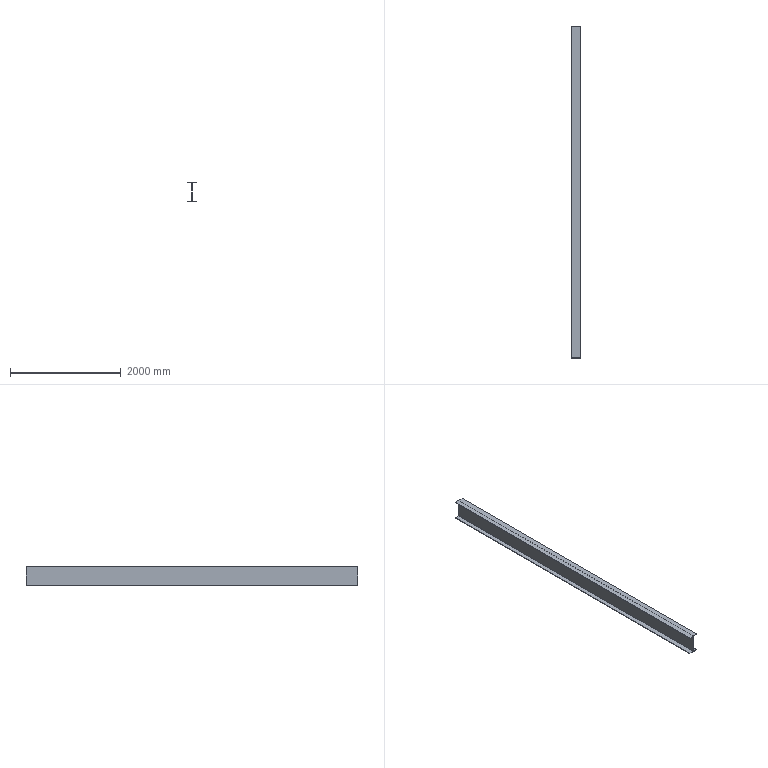Component | NX | ZHIJIA5 | 1 solid | 14 faces | box 175 x 6000 x 350 mm | volume 40800000 mm3 | plane 14
STEP:
#1=CARTESIAN_POINT('',(0.,0.,0.));
#2=DIRECTION('',(0.,0.,1.));
#3=DIRECTION('',(1.,0.,0.));
#4=AXIS2_PLACEMENT_3D('',#1,#2,#3);
#5=CARTESIAN_POINT('',(-2587.5,3000.,459.553));
#6=VERTEX_POINT('',#5);
#7=CARTESIAN_POINT('',(-2587.5,3000.,449.553));
#8=VERTEX_POINT('',#7);
#9=CARTESIAN_POINT('',(-2587.5,3000.,459.553));
#10=DIRECTION('',(-0.,0.,-1.));
#11=VECTOR('',#10,1.);
#12=LINE('',#9,#11);
#13=CARTESIAN_POINT('',(-2587.5,-3000.,459.553));
#14=DIRECTION('',(1.,0.,-0.));
#15=DIRECTION('',(0.,0.,1.));
#16=AXIS2_PLACEMENT_3D('',#13,#14,#15);
#17=PLANE('',#16);
#18=CARTESIAN_POINT('',(0.,-6000.));
#19=DIRECTION('',(-1.,0.));
#20=VECTOR('',#19,1.);
#21=LINE('',#18,#20);
#22=(GEOMETRIC_REPRESENTATION_CONTEXT(2)PARAMETRIC_REPRESENTATION_CONTEXT()REPRESENTATION_CONTEXT('',''));
#23=DEFINITIONAL_REPRESENTATION('',(#21),#22);
#24=PCURVE('',#17,#23);
#25=CARTESIAN_POINT('',(-2587.5,3000.,449.553));
#26=DIRECTION('',(0.,-1.,0.));
#27=DIRECTION('',(1.,0.,0.));
#28=AXIS2_PLACEMENT_3D('',#25,#26,#27);
#29=PLANE('',#28);
#30=CARTESIAN_POINT('',(0.,10.));
#31=DIRECTION('',(-0.,-1.));
#32=VECTOR('',#31,1.);
#33=LINE('',#30,#32);
#34=(GEOMETRIC_REPRESENTATION_CONTEXT(2)PARAMETRIC_REPRESENTATION_CONTEXT()REPRESENTATION_CONTEXT('',''));
#35=DEFINITIONAL_REPRESENTATION('',(#33),#34);
#36=PCURVE('',#29,#35);
#37=SURFACE_CURVE('',#12,(#24,#36),.PCURVE_S1.);
#38=EDGE_CURVE('',#6,#8,#37,.T.);
#39=ORIENTED_EDGE('',*,*,#38,.T.);
#40=CARTESIAN_POINT('',(-2587.5,-3000.,449.553));
#41=VERTEX_POINT('',#40);
#42=CARTESIAN_POINT('',(-2587.5,-3000.,449.553));
#43=DIRECTION('',(0.,1.,0.));
#44=VECTOR('',#43,1.);
#45=LINE('',#42,#44);
#46=CARTESIAN_POINT('',(-10.,0.));
#47=DIRECTION('',(0.,-1.));
#48=VECTOR('',#47,1.);
#49=LINE('',#46,#48);
#50=(GEOMETRIC_REPRESENTATION_CONTEXT(2)PARAMETRIC_REPRESENTATION_CONTEXT()REPRESENTATION_CONTEXT('',''));
#51=DEFINITIONAL_REPRESENTATION('',(#49),#50);
#52=PCURVE('',#17,#51);
#53=CARTESIAN_POINT('',(-2587.5,-3000.,449.553));
#54=DIRECTION('',(0.,0.,1.));
#55=DIRECTION('',(0.,-1.,0.));
#56=AXIS2_PLACEMENT_3D('',#53,#54,#55);
#57=PLANE('',#56);
#58=CARTESIAN_POINT('',(0.,0.));
#59=DIRECTION('',(-1.,0.));
#60=VECTOR('',#59,1.);
#61=LINE('',#58,#60);
#62=(GEOMETRIC_REPRESENTATION_CONTEXT(2)PARAMETRIC_REPRESENTATION_CONTEXT()REPRESENTATION_CONTEXT('',''));
#63=DEFINITIONAL_REPRESENTATION('',(#61),#62);
#64=PCURVE('',#57,#63);
#65=SURFACE_CURVE('',#45,(#52,#64),.PCURVE_S1.);
#66=EDGE_CURVE('',#41,#8,#65,.T.);
#67=ORIENTED_EDGE('',*,*,#66,.F.);
#68=CARTESIAN_POINT('',(-2587.5,-3000.,459.553));
#69=VERTEX_POINT('',#68);
#70=CARTESIAN_POINT('',(-2587.5,-3000.,459.553));
#71=DIRECTION('',(-0.,0.,-1.));
#72=VECTOR('',#71,1.);
#73=LINE('',#70,#72);
#74=CARTESIAN_POINT('',(0.,0.));
#75=DIRECTION('',(-1.,0.));
#76=VECTOR('',#75,1.);
#77=LINE('',#74,#76);
#78=(GEOMETRIC_REPRESENTATION_CONTEXT(2)PARAMETRIC_REPRESENTATION_CONTEXT()REPRESENTATION_CONTEXT('',''));
#79=DEFINITIONAL_REPRESENTATION('',(#77),#78);
#80=PCURVE('',#17,#79);
#81=CARTESIAN_POINT('',(-2587.5,-3000.,449.553));
#82=DIRECTION('',(0.,-1.,0.));
#83=DIRECTION('',(1.,0.,0.));
#84=AXIS2_PLACEMENT_3D('',#81,#82,#83);
#85=PLANE('',#84);
#86=CARTESIAN_POINT('',(0.,10.));
#87=DIRECTION('',(-0.,-1.));
#88=VECTOR('',#87,1.);
#89=LINE('',#86,#88);
#90=(GEOMETRIC_REPRESENTATION_CONTEXT(2)PARAMETRIC_REPRESENTATION_CONTEXT()REPRESENTATION_CONTEXT('',''));
#91=DEFINITIONAL_REPRESENTATION('',(#89),#90);
#92=PCURVE('',#85,#91);
#93=SURFACE_CURVE('',#73,(#80,#92),.PCURVE_S1.);
#94=EDGE_CURVE('',#69,#41,#93,.T.);
#95=ORIENTED_EDGE('',*,*,#94,.F.);
#96=CARTESIAN_POINT('',(-2587.5,-3000.,459.553));
#97=DIRECTION('',(0.,1.,0.));
#98=VECTOR('',#97,1.);
#99=LINE('',#96,#98);
#100=CARTESIAN_POINT('',(0.,0.));
#101=DIRECTION('',(0.,-1.));
#102=VECTOR('',#101,1.);
#103=LINE('',#100,#102);
#104=(GEOMETRIC_REPRESENTATION_CONTEXT(2)PARAMETRIC_REPRESENTATION_CONTEXT()REPRESENTATION_CONTEXT('',''));
#105=DEFINITIONAL_REPRESENTATION('',(#103),#104);
#106=PCURVE('',#17,#105);
#107=CARTESIAN_POINT('',(-2505.,-3000.,459.553));
#108=DIRECTION('',(0.,0.,-1.));
#109=DIRECTION('',(0.,1.,0.));
#110=AXIS2_PLACEMENT_3D('',#107,#108,#109);
#111=PLANE('',#110);
#112=CARTESIAN_POINT('',(0.,-82.5));
#113=DIRECTION('',(1.,0.));
#114=VECTOR('',#113,1.);
#115=LINE('',#112,#114);
#116=(GEOMETRIC_REPRESENTATION_CONTEXT(2)PARAMETRIC_REPRESENTATION_CONTEXT()REPRESENTATION_CONTEXT('',''));
#117=DEFINITIONAL_REPRESENTATION('',(#115),#116);
#118=PCURVE('',#111,#117);
#119=SURFACE_CURVE('',#99,(#106,#118),.PCURVE_S1.);
#120=EDGE_CURVE('',#69,#6,#119,.T.);
#121=ORIENTED_EDGE('',*,*,#120,.T.);
#122=EDGE_LOOP('',(#39,#67,#95,#121));
#123=FACE_BOUND('',#122,.T.);
#124=ADVANCED_FACE('',(#123),#17,.F.);
#125=CARTESIAN_POINT('',(-2412.5,3000.,449.553));
#126=VERTEX_POINT('',#125);
#127=CARTESIAN_POINT('',(-2587.5,3000.,449.553));
#128=DIRECTION('',(1.,0.,0.));
#129=VECTOR('',#128,1.);
#130=LINE('',#127,#129);
#131=CARTESIAN_POINT('',(-6000.,0.));
#132=DIRECTION('',(0.,1.));
#133=VECTOR('',#132,1.);
#134=LINE('',#131,#133);
#135=(GEOMETRIC_REPRESENTATION_CONTEXT(2)PARAMETRIC_REPRESENTATION_CONTEXT()REPRESENTATION_CONTEXT('',''));
#136=DEFINITIONAL_REPRESENTATION('',(#134),#135);
#137=PCURVE('',#57,#136);
#138=CARTESIAN_POINT('',(0.,0.));
#139=DIRECTION('',(1.,0.));
#140=VECTOR('',#139,1.);
#141=LINE('',#138,#140);
#142=(GEOMETRIC_REPRESENTATION_CONTEXT(2)PARAMETRIC_REPRESENTATION_CONTEXT()REPRESENTATION_CONTEXT('',''));
#143=DEFINITIONAL_REPRESENTATION('',(#141),#142);
#144=PCURVE('',#29,#143);
#145=SURFACE_CURVE('',#130,(#137,#144),.PCURVE_S1.);
#146=EDGE_CURVE('',#8,#126,#145,.T.);
#147=ORIENTED_EDGE('',*,*,#146,.T.);
#148=CARTESIAN_POINT('',(-2412.5,-3000.,449.553));
#149=VERTEX_POINT('',#148);
#150=CARTESIAN_POINT('',(-2412.5,-3000.,449.553));
#151=DIRECTION('',(0.,1.,0.));
#152=VECTOR('',#151,1.);
#153=LINE('',#150,#152);
#154=CARTESIAN_POINT('',(0.,175.));
#155=DIRECTION('',(-1.,0.));
#156=VECTOR('',#155,1.);
#157=LINE('',#154,#156);
#158=(GEOMETRIC_REPRESENTATION_CONTEXT(2)PARAMETRIC_REPRESENTATION_CONTEXT()REPRESENTATION_CONTEXT('',''));
#159=DEFINITIONAL_REPRESENTATION('',(#157),#158);
#160=PCURVE('',#57,#159);
#161=CARTESIAN_POINT('',(-2412.5,-3000.,449.553));
#162=DIRECTION('',(-1.,0.,0.));
#163=DIRECTION('',(-0.,0.,-1.));
#164=AXIS2_PLACEMENT_3D('',#161,#162,#163);
#165=PLANE('',#164);
#166=CARTESIAN_POINT('',(-0.,0.));
#167=DIRECTION('',(0.,-1.));
#168=VECTOR('',#167,1.);
#169=LINE('',#166,#168);
#170=(GEOMETRIC_REPRESENTATION_CONTEXT(2)PARAMETRIC_REPRESENTATION_CONTEXT()REPRESENTATION_CONTEXT('',''));
#171=DEFINITIONAL_REPRESENTATION('',(#169),#170);
#172=PCURVE('',#165,#171);
#173=SURFACE_CURVE('',#153,(#160,#172),.PCURVE_S1.);
#174=EDGE_CURVE('',#149,#126,#173,.T.);
#175=ORIENTED_EDGE('',*,*,#174,.F.);
#176=CARTESIAN_POINT('',(-2587.5,-3000.,449.553));
#177=DIRECTION('',(1.,0.,0.));
#178=VECTOR('',#177,1.);
#179=LINE('',#176,#178);
#180=CARTESIAN_POINT('',(0.,0.));
#181=DIRECTION('',(0.,1.));
#182=VECTOR('',#181,1.);
#183=LINE('',#180,#182);
#184=(GEOMETRIC_REPRESENTATION_CONTEXT(2)PARAMETRIC_REPRESENTATION_CONTEXT()REPRESENTATION_CONTEXT('',''));
#185=DEFINITIONAL_REPRESENTATION('',(#183),#184);
#186=PCURVE('',#57,#185);
#187=CARTESIAN_POINT('',(0.,0.));
#188=DIRECTION('',(1.,0.));
#189=VECTOR('',#188,1.);
#190=LINE('',#187,#189);
#191=(GEOMETRIC_REPRESENTATION_CONTEXT(2)PARAMETRIC_REPRESENTATION_CONTEXT()REPRESENTATION_CONTEXT('',''));
#192=DEFINITIONAL_REPRESENTATION('',(#190),#191);
#193=PCURVE('',#85,#192);
#194=SURFACE_CURVE('',#179,(#186,#193),.PCURVE_S1.);
#195=EDGE_CURVE('',#41,#149,#194,.T.);
#196=ORIENTED_EDGE('',*,*,#195,.F.);
#197=ORIENTED_EDGE('',*,*,#66,.T.);
#198=EDGE_LOOP('',(#147,#175,#196,#197));
#199=FACE_BOUND('',#198,.T.);
#200=ADVANCED_FACE('',(#199),#57,.F.);
#201=CARTESIAN_POINT('',(-2412.5,3000.,459.553));
#202=VERTEX_POINT('',#201);
#203=CARTESIAN_POINT('',(-2412.5,3000.,449.553));
#204=DIRECTION('',(0.,0.,1.));
#205=VECTOR('',#204,1.);
#206=LINE('',#203,#205);
#207=CARTESIAN_POINT('',(0.,-6000.));
#208=DIRECTION('',(-1.,0.));
#209=VECTOR('',#208,1.);
#210=LINE('',#207,#209);
#211=(GEOMETRIC_REPRESENTATION_CONTEXT(2)PARAMETRIC_REPRESENTATION_CONTEXT()REPRESENTATION_CONTEXT('',''));
#212=DEFINITIONAL_REPRESENTATION('',(#210),#211);
#213=PCURVE('',#165,#212);
#214=CARTESIAN_POINT('',(175.,-0.));
#215=DIRECTION('',(0.,1.));
#216=VECTOR('',#215,1.);
#217=LINE('',#214,#216);
#218=(GEOMETRIC_REPRESENTATION_CONTEXT(2)PARAMETRIC_REPRESENTATION_CONTEXT()REPRESENTATION_CONTEXT('',''));
#219=DEFINITIONAL_REPRESENTATION('',(#217),#218);
#220=PCURVE('',#29,#219);
#221=SURFACE_CURVE('',#206,(#213,#220),.PCURVE_S1.);
#222=EDGE_CURVE('',#126,#202,#221,.T.);
#223=ORIENTED_EDGE('',*,*,#222,.T.);
#224=CARTESIAN_POINT('',(-2412.5,-3000.,459.553));
#225=VERTEX_POINT('',#224);
#226=CARTESIAN_POINT('',(-2412.5,-3000.,459.553));
#227=DIRECTION('',(0.,1.,0.));
#228=VECTOR('',#227,1.);
#229=LINE('',#226,#228);
#230=CARTESIAN_POINT('',(-10.,0.));
#231=DIRECTION('',(0.,-1.));
#232=VECTOR('',#231,1.);
#233=LINE('',#230,#232);
#234=(GEOMETRIC_REPRESENTATION_CONTEXT(2)PARAMETRIC_REPRESENTATION_CONTEXT()REPRESENTATION_CONTEXT('',''));
#235=DEFINITIONAL_REPRESENTATION('',(#233),#234);
#236=PCURVE('',#165,#235);
#237=CARTESIAN_POINT('',(-2412.5,-3000.,459.553));
#238=DIRECTION('',(0.,0.,-1.));
#239=DIRECTION('',(0.,1.,0.));
#240=AXIS2_PLACEMENT_3D('',#237,#238,#239);
#241=PLANE('',#240);
#242=CARTESIAN_POINT('',(0.,0.));
#243=DIRECTION('',(1.,0.));
#244=VECTOR('',#243,1.);
#245=LINE('',#242,#244);
#246=(GEOMETRIC_REPRESENTATION_CONTEXT(2)PARAMETRIC_REPRESENTATION_CONTEXT()REPRESENTATION_CONTEXT('',''));
#247=DEFINITIONAL_REPRESENTATION('',(#245),#246);
#248=PCURVE('',#241,#247);
#249=SURFACE_CURVE('',#229,(#236,#248),.PCURVE_S1.);
#250=EDGE_CURVE('',#225,#202,#249,.T.);
#251=ORIENTED_EDGE('',*,*,#250,.F.);
#252=CARTESIAN_POINT('',(-2412.5,-3000.,449.553));
#253=DIRECTION('',(0.,0.,1.));
#254=VECTOR('',#253,1.);
#255=LINE('',#252,#254);
#256=CARTESIAN_POINT('',(0.,0.));
#257=DIRECTION('',(-1.,0.));
#258=VECTOR('',#257,1.);
#259=LINE('',#256,#258);
#260=(GEOMETRIC_REPRESENTATION_CONTEXT(2)PARAMETRIC_REPRESENTATION_CONTEXT()REPRESENTATION_CONTEXT('',''));
#261=DEFINITIONAL_REPRESENTATION('',(#259),#260);
#262=PCURVE('',#165,#261);
#263=CARTESIAN_POINT('',(175.,-0.));
#264=DIRECTION('',(0.,1.));
#265=VECTOR('',#264,1.);
#266=LINE('',#263,#265);
#267=(GEOMETRIC_REPRESENTATION_CONTEXT(2)PARAMETRIC_REPRESENTATION_CONTEXT()REPRESENTATION_CONTEXT('',''));
#268=DEFINITIONAL_REPRESENTATION('',(#266),#267);
#269=PCURVE('',#85,#268);
#270=SURFACE_CURVE('',#255,(#262,#269),.PCURVE_S1.);
#271=EDGE_CURVE('',#149,#225,#270,.T.);
#272=ORIENTED_EDGE('',*,*,#271,.F.);
#273=ORIENTED_EDGE('',*,*,#174,.T.);
#274=EDGE_LOOP('',(#223,#251,#272,#273));
#275=FACE_BOUND('',#274,.T.);
#276=ADVANCED_FACE('',(#275),#165,.F.);
#277=CARTESIAN_POINT('',(-2495.,3000.,459.553));
#278=VERTEX_POINT('',#277);
#279=CARTESIAN_POINT('',(-2412.5,3000.,459.553));
#280=DIRECTION('',(-1.,0.,0.));
#281=VECTOR('',#280,1.);
#282=LINE('',#279,#281);
#283=CARTESIAN_POINT('',(6000.,0.));
#284=DIRECTION('',(0.,-1.));
#285=VECTOR('',#284,1.);
#286=LINE('',#283,#285);
#287=(GEOMETRIC_REPRESENTATION_CONTEXT(2)PARAMETRIC_REPRESENTATION_CONTEXT()REPRESENTATION_CONTEXT('',''));
#288=DEFINITIONAL_REPRESENTATION('',(#286),#287);
#289=PCURVE('',#241,#288);
#290=CARTESIAN_POINT('',(175.,10.));
#291=DIRECTION('',(-1.,0.));
#292=VECTOR('',#291,1.);
#293=LINE('',#290,#292);
#294=(GEOMETRIC_REPRESENTATION_CONTEXT(2)PARAMETRIC_REPRESENTATION_CONTEXT()REPRESENTATION_CONTEXT('',''));
#295=DEFINITIONAL_REPRESENTATION('',(#293),#294);
#296=PCURVE('',#29,#295);
#297=SURFACE_CURVE('',#282,(#289,#296),.PCURVE_S1.);
#298=EDGE_CURVE('',#202,#278,#297,.T.);
#299=ORIENTED_EDGE('',*,*,#298,.T.);
#300=CARTESIAN_POINT('',(-2495.,-3000.,459.553));
#301=VERTEX_POINT('',#300);
#302=CARTESIAN_POINT('',(-2495.,-3000.,459.553));
#303=DIRECTION('',(0.,1.,0.));
#304=VECTOR('',#303,1.);
#305=LINE('',#302,#304);
#306=CARTESIAN_POINT('',(0.,-82.5));
#307=DIRECTION('',(1.,0.));
#308=VECTOR('',#307,1.);
#309=LINE('',#306,#308);
#310=(GEOMETRIC_REPRESENTATION_CONTEXT(2)PARAMETRIC_REPRESENTATION_CONTEXT()REPRESENTATION_CONTEXT('',''));
#311=DEFINITIONAL_REPRESENTATION('',(#309),#310);
#312=PCURVE('',#241,#311);
#313=CARTESIAN_POINT('',(-2495.,-3000.,459.553));
#314=DIRECTION('',(-1.,0.,0.));
#315=DIRECTION('',(-0.,0.,-1.));
#316=AXIS2_PLACEMENT_3D('',#313,#314,#315);
#317=PLANE('',#316);
#318=CARTESIAN_POINT('',(0.,0.));
#319=DIRECTION('',(0.,-1.));
#320=VECTOR('',#319,1.);
#321=LINE('',#318,#320);
#322=(GEOMETRIC_REPRESENTATION_CONTEXT(2)PARAMETRIC_REPRESENTATION_CONTEXT()REPRESENTATION_CONTEXT('',''));
#323=DEFINITIONAL_REPRESENTATION('',(#321),#322);
#324=PCURVE('',#317,#323);
#325=SURFACE_CURVE('',#305,(#312,#324),.PCURVE_S1.);
#326=EDGE_CURVE('',#301,#278,#325,.T.);
#327=ORIENTED_EDGE('',*,*,#326,.F.);
#328=CARTESIAN_POINT('',(-2412.5,-3000.,459.553));
#329=DIRECTION('',(-1.,0.,0.));
#330=VECTOR('',#329,1.);
#331=LINE('',#328,#330);
#332=CARTESIAN_POINT('',(0.,0.));
#333=DIRECTION('',(0.,-1.));
#334=VECTOR('',#333,1.);
#335=LINE('',#332,#334);
#336=(GEOMETRIC_REPRESENTATION_CONTEXT(2)PARAMETRIC_REPRESENTATION_CONTEXT()REPRESENTATION_CONTEXT('',''));
#337=DEFINITIONAL_REPRESENTATION('',(#335),#336);
#338=PCURVE('',#241,#337);
#339=CARTESIAN_POINT('',(175.,10.));
#340=DIRECTION('',(-1.,0.));
#341=VECTOR('',#340,1.);
#342=LINE('',#339,#341);
#343=(GEOMETRIC_REPRESENTATION_CONTEXT(2)PARAMETRIC_REPRESENTATION_CONTEXT()REPRESENTATION_CONTEXT('',''));
#344=DEFINITIONAL_REPRESENTATION('',(#342),#343);
#345=PCURVE('',#85,#344);
#346=SURFACE_CURVE('',#331,(#338,#345),.PCURVE_S1.);
#347=EDGE_CURVE('',#225,#301,#346,.T.);
#348=ORIENTED_EDGE('',*,*,#347,.F.);
#349=ORIENTED_EDGE('',*,*,#250,.T.);
#350=EDGE_LOOP('',(#299,#327,#348,#349));
#351=FACE_BOUND('',#350,.T.);
#352=ADVANCED_FACE('',(#351),#241,.F.);
#353=CARTESIAN_POINT('',(-2495.,3000.,789.553));
#354=VERTEX_POINT('',#353);
#355=CARTESIAN_POINT('',(-2495.,3000.,459.553));
#356=DIRECTION('',(0.,0.,1.));
#357=VECTOR('',#356,1.);
#358=LINE('',#355,#357);
#359=CARTESIAN_POINT('',(0.,-6000.));
#360=DIRECTION('',(-1.,0.));
#361=VECTOR('',#360,1.);
#362=LINE('',#359,#361);
#363=(GEOMETRIC_REPRESENTATION_CONTEXT(2)PARAMETRIC_REPRESENTATION_CONTEXT()REPRESENTATION_CONTEXT('',''));
#364=DEFINITIONAL_REPRESENTATION('',(#362),#363);
#365=PCURVE('',#317,#364);
#366=CARTESIAN_POINT('',(92.5,10.));
#367=DIRECTION('',(0.,1.));
#368=VECTOR('',#367,1.);
#369=LINE('',#366,#368);
#370=(GEOMETRIC_REPRESENTATION_CONTEXT(2)PARAMETRIC_REPRESENTATION_CONTEXT()REPRESENTATION_CONTEXT('',''));
#371=DEFINITIONAL_REPRESENTATION('',(#369),#370);
#372=PCURVE('',#29,#371);
#373=SURFACE_CURVE('',#358,(#365,#372),.PCURVE_S1.);
#374=EDGE_CURVE('',#278,#354,#373,.T.);
#375=ORIENTED_EDGE('',*,*,#374,.T.);
#376=CARTESIAN_POINT('',(-2495.,-3000.,789.553));
#377=VERTEX_POINT('',#376);
#378=CARTESIAN_POINT('',(-2495.,-3000.,789.553));
#379=DIRECTION('',(0.,1.,0.));
#380=VECTOR('',#379,1.);
#381=LINE('',#378,#380);
#382=CARTESIAN_POINT('',(-330.,0.));
#383=DIRECTION('',(0.,-1.));
#384=VECTOR('',#383,1.);
#385=LINE('',#382,#384);
#386=(GEOMETRIC_REPRESENTATION_CONTEXT(2)PARAMETRIC_REPRESENTATION_CONTEXT()REPRESENTATION_CONTEXT('',''));
#387=DEFINITIONAL_REPRESENTATION('',(#385),#386);
#388=PCURVE('',#317,#387);
#389=CARTESIAN_POINT('',(-2495.,-3000.,789.553));
#390=DIRECTION('',(0.,0.,1.));
#391=DIRECTION('',(0.,-1.,0.));
#392=AXIS2_PLACEMENT_3D('',#389,#390,#391);
#393=PLANE('',#392);
#394=CARTESIAN_POINT('',(0.,0.));
#395=DIRECTION('',(-1.,0.));
#396=VECTOR('',#395,1.);
#397=LINE('',#394,#396);
#398=(GEOMETRIC_REPRESENTATION_CONTEXT(2)PARAMETRIC_REPRESENTATION_CONTEXT()REPRESENTATION_CONTEXT('',''));
#399=DEFINITIONAL_REPRESENTATION('',(#397),#398);
#400=PCURVE('',#393,#399);
#401=SURFACE_CURVE('',#381,(#388,#400),.PCURVE_S1.);
#402=EDGE_CURVE('',#377,#354,#401,.T.);
#403=ORIENTED_EDGE('',*,*,#402,.F.);
#404=CARTESIAN_POINT('',(-2495.,-3000.,459.553));
#405=DIRECTION('',(0.,0.,1.));
#406=VECTOR('',#405,1.);
#407=LINE('',#404,#406);
#408=CARTESIAN_POINT('',(0.,0.));
#409=DIRECTION('',(-1.,0.));
#410=VECTOR('',#409,1.);
#411=LINE('',#408,#410);
#412=(GEOMETRIC_REPRESENTATION_CONTEXT(2)PARAMETRIC_REPRESENTATION_CONTEXT()REPRESENTATION_CONTEXT('',''));
#413=DEFINITIONAL_REPRESENTATION('',(#411),#412);
#414=PCURVE('',#317,#413);
#415=CARTESIAN_POINT('',(92.5,10.));
#416=DIRECTION('',(0.,1.));
#417=VECTOR('',#416,1.);
#418=LINE('',#415,#417);
#419=(GEOMETRIC_REPRESENTATION_CONTEXT(2)PARAMETRIC_REPRESENTATION_CONTEXT()REPRESENTATION_CONTEXT('',''));
#420=DEFINITIONAL_REPRESENTATION('',(#418),#419);
#421=PCURVE('',#85,#420);
#422=SURFACE_CURVE('',#407,(#414,#421),.PCURVE_S1.);
#423=EDGE_CURVE('',#301,#377,#422,.T.);
#424=ORIENTED_EDGE('',*,*,#423,.F.);
#425=ORIENTED_EDGE('',*,*,#326,.T.);
#426=EDGE_LOOP('',(#375,#403,#424,#425));
#427=FACE_BOUND('',#426,.T.);
#428=ADVANCED_FACE('',(#427),#317,.F.);
#429=CARTESIAN_POINT('',(-2412.5,3000.,789.553));
#430=VERTEX_POINT('',#429);
#431=CARTESIAN_POINT('',(-2495.,3000.,789.553));
#432=DIRECTION('',(1.,0.,0.));
#433=VECTOR('',#432,1.);
#434=LINE('',#431,#433);
#435=CARTESIAN_POINT('',(-6000.,0.));
#436=DIRECTION('',(0.,1.));
#437=VECTOR('',#436,1.);
#438=LINE('',#435,#437);
#439=(GEOMETRIC_REPRESENTATION_CONTEXT(2)PARAMETRIC_REPRESENTATION_CONTEXT()REPRESENTATION_CONTEXT('',''));
#440=DEFINITIONAL_REPRESENTATION('',(#438),#439);
#441=PCURVE('',#393,#440);
#442=CARTESIAN_POINT('',(92.5,340.));
#443=DIRECTION('',(1.,0.));
#444=VECTOR('',#443,1.);
#445=LINE('',#442,#444);
#446=(GEOMETRIC_REPRESENTATION_CONTEXT(2)PARAMETRIC_REPRESENTATION_CONTEXT()REPRESENTATION_CONTEXT('',''));
#447=DEFINITIONAL_REPRESENTATION('',(#445),#446);
#448=PCURVE('',#29,#447);
#449=SURFACE_CURVE('',#434,(#441,#448),.PCURVE_S1.);
#450=EDGE_CURVE('',#354,#430,#449,.T.);
#451=ORIENTED_EDGE('',*,*,#450,.T.);
#452=CARTESIAN_POINT('',(-2412.5,-3000.,789.553));
#453=VERTEX_POINT('',#452);
#454=CARTESIAN_POINT('',(-2412.5,-3000.,789.553));
#455=DIRECTION('',(0.,1.,0.));
#456=VECTOR('',#455,1.);
#457=LINE('',#454,#456);
#458=CARTESIAN_POINT('',(0.,82.5));
#459=DIRECTION('',(-1.,0.));
#460=VECTOR('',#459,1.);
#461=LINE('',#458,#460);
#462=(GEOMETRIC_REPRESENTATION_CONTEXT(2)PARAMETRIC_REPRESENTATION_CONTEXT()REPRESENTATION_CONTEXT('',''));
#463=DEFINITIONAL_REPRESENTATION('',(#461),#462);
#464=PCURVE('',#393,#463);
#465=CARTESIAN_POINT('',(-2412.5,-3000.,789.553));
#466=DIRECTION('',(-1.,0.,0.));
#467=DIRECTION('',(-0.,0.,-1.));
#468=AXIS2_PLACEMENT_3D('',#465,#466,#467);
#469=PLANE('',#468);
#470=CARTESIAN_POINT('',(0.,0.));
#471=DIRECTION('',(0.,-1.));
#472=VECTOR('',#471,1.);
#473=LINE('',#470,#472);
#474=(GEOMETRIC_REPRESENTATION_CONTEXT(2)PARAMETRIC_REPRESENTATION_CONTEXT()REPRESENTATION_CONTEXT('',''));
#475=DEFINITIONAL_REPRESENTATION('',(#473),#474);
#476=PCURVE('',#469,#475);
#477=SURFACE_CURVE('',#457,(#464,#476),.PCURVE_S1.);
#478=EDGE_CURVE('',#453,#430,#477,.T.);
#479=ORIENTED_EDGE('',*,*,#478,.F.);
#480=CARTESIAN_POINT('',(-2495.,-3000.,789.553));
#481=DIRECTION('',(1.,0.,0.));
#482=VECTOR('',#481,1.);
#483=LINE('',#480,#482);
#484=CARTESIAN_POINT('',(0.,0.));
#485=DIRECTION('',(0.,1.));
#486=VECTOR('',#485,1.);
#487=LINE('',#484,#486);
#488=(GEOMETRIC_REPRESENTATION_CONTEXT(2)PARAMETRIC_REPRESENTATION_CONTEXT()REPRESENTATION_CONTEXT('',''));
#489=DEFINITIONAL_REPRESENTATION('',(#487),#488);
#490=PCURVE('',#393,#489);
#491=CARTESIAN_POINT('',(92.5,340.));
#492=DIRECTION('',(1.,0.));
#493=VECTOR('',#492,1.);
#494=LINE('',#491,#493);
#495=(GEOMETRIC_REPRESENTATION_CONTEXT(2)PARAMETRIC_REPRESENTATION_CONTEXT()REPRESENTATION_CONTEXT('',''));
#496=DEFINITIONAL_REPRESENTATION('',(#494),#495);
#497=PCURVE('',#85,#496);
#498=SURFACE_CURVE('',#483,(#490,#497),.PCURVE_S1.);
#499=EDGE_CURVE('',#377,#453,#498,.T.);
#500=ORIENTED_EDGE('',*,*,#499,.F.);
#501=ORIENTED_EDGE('',*,*,#402,.T.);
#502=EDGE_LOOP('',(#451,#479,#500,#501));
#503=FACE_BOUND('',#502,.T.);
#504=ADVANCED_FACE('',(#503),#393,.F.);
#505=CARTESIAN_POINT('',(-2412.5,3000.,799.553));
#506=VERTEX_POINT('',#505);
#507=CARTESIAN_POINT('',(-2412.5,3000.,789.553));
#508=DIRECTION('',(0.,0.,1.));
#509=VECTOR('',#508,1.);
#510=LINE('',#507,#509);
#511=CARTESIAN_POINT('',(0.,-6000.));
#512=DIRECTION('',(-1.,0.));
#513=VECTOR('',#512,1.);
#514=LINE('',#511,#513);
#515=(GEOMETRIC_REPRESENTATION_CONTEXT(2)PARAMETRIC_REPRESENTATION_CONTEXT()REPRESENTATION_CONTEXT('',''));
#516=DEFINITIONAL_REPRESENTATION('',(#514),#515);
#517=PCURVE('',#469,#516);
#518=CARTESIAN_POINT('',(175.,340.));
#519=DIRECTION('',(0.,1.));
#520=VECTOR('',#519,1.);
#521=LINE('',#518,#520);
#522=(GEOMETRIC_REPRESENTATION_CONTEXT(2)PARAMETRIC_REPRESENTATION_CONTEXT()REPRESENTATION_CONTEXT('',''));
#523=DEFINITIONAL_REPRESENTATION('',(#521),#522);
#524=PCURVE('',#29,#523);
#525=SURFACE_CURVE('',#510,(#517,#524),.PCURVE_S1.);
#526=EDGE_CURVE('',#430,#506,#525,.T.);
#527=ORIENTED_EDGE('',*,*,#526,.T.);
#528=CARTESIAN_POINT('',(-2412.5,-3000.,799.553));
#529=VERTEX_POINT('',#528);
#530=CARTESIAN_POINT('',(-2412.5,-3000.,799.553));
#531=DIRECTION('',(0.,1.,0.));
#532=VECTOR('',#531,1.);
#533=LINE('',#530,#532);
#534=CARTESIAN_POINT('',(-10.,0.));
#535=DIRECTION('',(0.,-1.));
#536=VECTOR('',#535,1.);
#537=LINE('',#534,#536);
#538=(GEOMETRIC_REPRESENTATION_CONTEXT(2)PARAMETRIC_REPRESENTATION_CONTEXT()REPRESENTATION_CONTEXT('',''));
#539=DEFINITIONAL_REPRESENTATION('',(#537),#538);
#540=PCURVE('',#469,#539);
#541=CARTESIAN_POINT('',(-2412.5,-3000.,799.553));
#542=DIRECTION('',(0.,0.,-1.));
#543=DIRECTION('',(0.,1.,0.));
#544=AXIS2_PLACEMENT_3D('',#541,#542,#543);
#545=PLANE('',#544);
#546=CARTESIAN_POINT('',(0.,0.));
#547=DIRECTION('',(1.,0.));
#548=VECTOR('',#547,1.);
#549=LINE('',#546,#548);
#550=(GEOMETRIC_REPRESENTATION_CONTEXT(2)PARAMETRIC_REPRESENTATION_CONTEXT()REPRESENTATION_CONTEXT('',''));
#551=DEFINITIONAL_REPRESENTATION('',(#549),#550);
#552=PCURVE('',#545,#551);
#553=SURFACE_CURVE('',#533,(#540,#552),.PCURVE_S1.);
#554=EDGE_CURVE('',#529,#506,#553,.T.);
#555=ORIENTED_EDGE('',*,*,#554,.F.);
#556=CARTESIAN_POINT('',(-2412.5,-3000.,789.553));
#557=DIRECTION('',(0.,0.,1.));
#558=VECTOR('',#557,1.);
#559=LINE('',#556,#558);
#560=CARTESIAN_POINT('',(0.,0.));
#561=DIRECTION('',(-1.,0.));
#562=VECTOR('',#561,1.);
#563=LINE('',#560,#562);
#564=(GEOMETRIC_REPRESENTATION_CONTEXT(2)PARAMETRIC_REPRESENTATION_CONTEXT()REPRESENTATION_CONTEXT('',''));
#565=DEFINITIONAL_REPRESENTATION('',(#563),#564);
#566=PCURVE('',#469,#565);
#567=CARTESIAN_POINT('',(175.,340.));
#568=DIRECTION('',(0.,1.));
#569=VECTOR('',#568,1.);
#570=LINE('',#567,#569);
#571=(GEOMETRIC_REPRESENTATION_CONTEXT(2)PARAMETRIC_REPRESENTATION_CONTEXT()REPRESENTATION_CONTEXT('',''));
#572=DEFINITIONAL_REPRESENTATION('',(#570),#571);
#573=PCURVE('',#85,#572);
#574=SURFACE_CURVE('',#559,(#566,#573),.PCURVE_S1.);
#575=EDGE_CURVE('',#453,#529,#574,.T.);
#576=ORIENTED_EDGE('',*,*,#575,.F.);
#577=ORIENTED_EDGE('',*,*,#478,.T.);
#578=EDGE_LOOP('',(#527,#555,#576,#577));
#579=FACE_BOUND('',#578,.T.);
#580=ADVANCED_FACE('',(#579),#469,.F.);
#581=CARTESIAN_POINT('',(-2587.5,3000.,799.553));
#582=VERTEX_POINT('',#581);
#583=CARTESIAN_POINT('',(-2412.5,3000.,799.553));
#584=DIRECTION('',(-1.,0.,0.));
#585=VECTOR('',#584,1.);
#586=LINE('',#583,#585);
#587=CARTESIAN_POINT('',(6000.,0.));
#588=DIRECTION('',(0.,-1.));
#589=VECTOR('',#588,1.);
#590=LINE('',#587,#589);
#591=(GEOMETRIC_REPRESENTATION_CONTEXT(2)PARAMETRIC_REPRESENTATION_CONTEXT()REPRESENTATION_CONTEXT('',''));
#592=DEFINITIONAL_REPRESENTATION('',(#590),#591);
#593=PCURVE('',#545,#592);
#594=CARTESIAN_POINT('',(175.,350.));
#595=DIRECTION('',(-1.,0.));
#596=VECTOR('',#595,1.);
#597=LINE('',#594,#596);
#598=(GEOMETRIC_REPRESENTATION_CONTEXT(2)PARAMETRIC_REPRESENTATION_CONTEXT()REPRESENTATION_CONTEXT('',''));
#599=DEFINITIONAL_REPRESENTATION('',(#597),#598);
#600=PCURVE('',#29,#599);
#601=SURFACE_CURVE('',#586,(#593,#600),.PCURVE_S1.);
#602=EDGE_CURVE('',#506,#582,#601,.T.);
#603=ORIENTED_EDGE('',*,*,#602,.T.);
#604=CARTESIAN_POINT('',(-2587.5,-3000.,799.553));
#605=VERTEX_POINT('',#604);
#606=CARTESIAN_POINT('',(-2587.5,-3000.,799.553));
#607=DIRECTION('',(0.,1.,0.));
#608=VECTOR('',#607,1.);
#609=LINE('',#606,#608);
#610=CARTESIAN_POINT('',(0.,-175.));
#611=DIRECTION('',(1.,0.));
#612=VECTOR('',#611,1.);
#613=LINE('',#610,#612);
#614=(GEOMETRIC_REPRESENTATION_CONTEXT(2)PARAMETRIC_REPRESENTATION_CONTEXT()REPRESENTATION_CONTEXT('',''));
#615=DEFINITIONAL_REPRESENTATION('',(#613),#614);
#616=PCURVE('',#545,#615);
#617=CARTESIAN_POINT('',(-2587.5,-3000.,799.553));
#618=DIRECTION('',(1.,0.,-0.));
#619=DIRECTION('',(0.,0.,1.));
#620=AXIS2_PLACEMENT_3D('',#617,#618,#619);
#621=PLANE('',#620);
#622=CARTESIAN_POINT('',(0.,0.));
#623=DIRECTION('',(0.,-1.));
#624=VECTOR('',#623,1.);
#625=LINE('',#622,#624);
#626=(GEOMETRIC_REPRESENTATION_CONTEXT(2)PARAMETRIC_REPRESENTATION_CONTEXT()REPRESENTATION_CONTEXT('',''));
#627=DEFINITIONAL_REPRESENTATION('',(#625),#626);
#628=PCURVE('',#621,#627);
#629=SURFACE_CURVE('',#609,(#616,#628),.PCURVE_S1.);
#630=EDGE_CURVE('',#605,#582,#629,.T.);
#631=ORIENTED_EDGE('',*,*,#630,.F.);
#632=CARTESIAN_POINT('',(-2412.5,-3000.,799.553));
#633=DIRECTION('',(-1.,0.,0.));
#634=VECTOR('',#633,1.);
#635=LINE('',#632,#634);
#636=CARTESIAN_POINT('',(0.,0.));
#637=DIRECTION('',(0.,-1.));
#638=VECTOR('',#637,1.);
#639=LINE('',#636,#638);
#640=(GEOMETRIC_REPRESENTATION_CONTEXT(2)PARAMETRIC_REPRESENTATION_CONTEXT()REPRESENTATION_CONTEXT('',''));
#641=DEFINITIONAL_REPRESENTATION('',(#639),#640);
#642=PCURVE('',#545,#641);
#643=CARTESIAN_POINT('',(175.,350.));
#644=DIRECTION('',(-1.,0.));
#645=VECTOR('',#644,1.);
#646=LINE('',#643,#645);
#647=(GEOMETRIC_REPRESENTATION_CONTEXT(2)PARAMETRIC_REPRESENTATION_CONTEXT()REPRESENTATION_CONTEXT('',''));
#648=DEFINITIONAL_REPRESENTATION('',(#646),#647);
#649=PCURVE('',#85,#648);
#650=SURFACE_CURVE('',#635,(#642,#649),.PCURVE_S1.);
#651=EDGE_CURVE('',#529,#605,#650,.T.);
#652=ORIENTED_EDGE('',*,*,#651,.F.);
#653=ORIENTED_EDGE('',*,*,#554,.T.);
#654=EDGE_LOOP('',(#603,#631,#652,#653));
#655=FACE_BOUND('',#654,.T.);
#656=ADVANCED_FACE('',(#655),#545,.F.);
#657=CARTESIAN_POINT('',(-2587.5,3000.,789.553));
#658=VERTEX_POINT('',#657);
#659=CARTESIAN_POINT('',(-2587.5,3000.,799.553));
#660=DIRECTION('',(-0.,0.,-1.));
#661=VECTOR('',#660,1.);
#662=LINE('',#659,#661);
#663=CARTESIAN_POINT('',(0.,-6000.));
#664=DIRECTION('',(-1.,0.));
#665=VECTOR('',#664,1.);
#666=LINE('',#663,#665);
#667=(GEOMETRIC_REPRESENTATION_CONTEXT(2)PARAMETRIC_REPRESENTATION_CONTEXT()REPRESENTATION_CONTEXT('',''));
#668=DEFINITIONAL_REPRESENTATION('',(#666),#667);
#669=PCURVE('',#621,#668);
#670=CARTESIAN_POINT('',(0.,350.));
#671=DIRECTION('',(-0.,-1.));
#672=VECTOR('',#671,1.);
#673=LINE('',#670,#672);
#674=(GEOMETRIC_REPRESENTATION_CONTEXT(2)PARAMETRIC_REPRESENTATION_CONTEXT()REPRESENTATION_CONTEXT('',''));
#675=DEFINITIONAL_REPRESENTATION('',(#673),#674);
#676=PCURVE('',#29,#675);
#677=SURFACE_CURVE('',#662,(#669,#676),.PCURVE_S1.);
#678=EDGE_CURVE('',#582,#658,#677,.T.);
#679=ORIENTED_EDGE('',*,*,#678,.T.);
#680=CARTESIAN_POINT('',(-2587.5,-3000.,789.553));
#681=VERTEX_POINT('',#680);
#682=CARTESIAN_POINT('',(-2587.5,-3000.,789.553));
#683=DIRECTION('',(0.,1.,0.));
#684=VECTOR('',#683,1.);
#685=LINE('',#682,#684);
#686=CARTESIAN_POINT('',(-10.,0.));
#687=DIRECTION('',(0.,-1.));
#688=VECTOR('',#687,1.);
#689=LINE('',#686,#688);
#690=(GEOMETRIC_REPRESENTATION_CONTEXT(2)PARAMETRIC_REPRESENTATION_CONTEXT()REPRESENTATION_CONTEXT('',''));
#691=DEFINITIONAL_REPRESENTATION('',(#689),#690);
#692=PCURVE('',#621,#691);
#693=CARTESIAN_POINT('',(-2587.5,-3000.,789.553));
#694=DIRECTION('',(0.,0.,1.));
#695=DIRECTION('',(0.,-1.,0.));
#696=AXIS2_PLACEMENT_3D('',#693,#694,#695);
#697=PLANE('',#696);
#698=CARTESIAN_POINT('',(0.,0.));
#699=DIRECTION('',(-1.,0.));
#700=VECTOR('',#699,1.);
#701=LINE('',#698,#700);
#702=(GEOMETRIC_REPRESENTATION_CONTEXT(2)PARAMETRIC_REPRESENTATION_CONTEXT()REPRESENTATION_CONTEXT('',''));
#703=DEFINITIONAL_REPRESENTATION('',(#701),#702);
#704=PCURVE('',#697,#703);
#705=SURFACE_CURVE('',#685,(#692,#704),.PCURVE_S1.);
#706=EDGE_CURVE('',#681,#658,#705,.T.);
#707=ORIENTED_EDGE('',*,*,#706,.F.);
#708=CARTESIAN_POINT('',(-2587.5,-3000.,799.553));
#709=DIRECTION('',(-0.,0.,-1.));
#710=VECTOR('',#709,1.);
#711=LINE('',#708,#710);
#712=CARTESIAN_POINT('',(0.,0.));
#713=DIRECTION('',(-1.,0.));
#714=VECTOR('',#713,1.);
#715=LINE('',#712,#714);
#716=(GEOMETRIC_REPRESENTATION_CONTEXT(2)PARAMETRIC_REPRESENTATION_CONTEXT()REPRESENTATION_CONTEXT('',''));
#717=DEFINITIONAL_REPRESENTATION('',(#715),#716);
#718=PCURVE('',#621,#717);
#719=CARTESIAN_POINT('',(0.,350.));
#720=DIRECTION('',(-0.,-1.));
#721=VECTOR('',#720,1.);
#722=LINE('',#719,#721);
#723=(GEOMETRIC_REPRESENTATION_CONTEXT(2)PARAMETRIC_REPRESENTATION_CONTEXT()REPRESENTATION_CONTEXT('',''));
#724=DEFINITIONAL_REPRESENTATION('',(#722),#723);
#725=PCURVE('',#85,#724);
#726=SURFACE_CURVE('',#711,(#718,#725),.PCURVE_S1.);
#727=EDGE_CURVE('',#605,#681,#726,.T.);
#728=ORIENTED_EDGE('',*,*,#727,.F.);
#729=ORIENTED_EDGE('',*,*,#630,.T.);
#730=EDGE_LOOP('',(#679,#707,#728,#729));
#731=FACE_BOUND('',#730,.T.);
#732=ADVANCED_FACE('',(#731),#621,.F.);
#733=CARTESIAN_POINT('',(-2505.,3000.,789.553));
#734=VERTEX_POINT('',#733);
#735=CARTESIAN_POINT('',(-2587.5,3000.,789.553));
#736=DIRECTION('',(1.,0.,0.));
#737=VECTOR('',#736,1.);
#738=LINE('',#735,#737);
#739=CARTESIAN_POINT('',(-6000.,0.));
#740=DIRECTION('',(0.,1.));
#741=VECTOR('',#740,1.);
#742=LINE('',#739,#741);
#743=(GEOMETRIC_REPRESENTATION_CONTEXT(2)PARAMETRIC_REPRESENTATION_CONTEXT()REPRESENTATION_CONTEXT('',''));
#744=DEFINITIONAL_REPRESENTATION('',(#742),#743);
#745=PCURVE('',#697,#744);
#746=CARTESIAN_POINT('',(0.,340.));
#747=DIRECTION('',(1.,0.));
#748=VECTOR('',#747,1.);
#749=LINE('',#746,#748);
#750=(GEOMETRIC_REPRESENTATION_CONTEXT(2)PARAMETRIC_REPRESENTATION_CONTEXT()REPRESENTATION_CONTEXT('',''));
#751=DEFINITIONAL_REPRESENTATION('',(#749),#750);
#752=PCURVE('',#29,#751);
#753=SURFACE_CURVE('',#738,(#745,#752),.PCURVE_S1.);
#754=EDGE_CURVE('',#658,#734,#753,.T.);
#755=ORIENTED_EDGE('',*,*,#754,.T.);
#756=CARTESIAN_POINT('',(-2505.,-3000.,789.553));
#757=VERTEX_POINT('',#756);
#758=CARTESIAN_POINT('',(-2505.,-3000.,789.553));
#759=DIRECTION('',(0.,1.,0.));
#760=VECTOR('',#759,1.);
#761=LINE('',#758,#760);
#762=CARTESIAN_POINT('',(0.,82.5));
#763=DIRECTION('',(-1.,0.));
#764=VECTOR('',#763,1.);
#765=LINE('',#762,#764);
#766=(GEOMETRIC_REPRESENTATION_CONTEXT(2)PARAMETRIC_REPRESENTATION_CONTEXT()REPRESENTATION_CONTEXT('',''));
#767=DEFINITIONAL_REPRESENTATION('',(#765),#766);
#768=PCURVE('',#697,#767);
#769=CARTESIAN_POINT('',(-2505.,-3000.,789.553));
#770=DIRECTION('',(1.,0.,-0.));
#771=DIRECTION('',(0.,0.,1.));
#772=AXIS2_PLACEMENT_3D('',#769,#770,#771);
#773=PLANE('',#772);
#774=CARTESIAN_POINT('',(0.,0.));
#775=DIRECTION('',(0.,-1.));
#776=VECTOR('',#775,1.);
#777=LINE('',#774,#776);
#778=(GEOMETRIC_REPRESENTATION_CONTEXT(2)PARAMETRIC_REPRESENTATION_CONTEXT()REPRESENTATION_CONTEXT('',''));
#779=DEFINITIONAL_REPRESENTATION('',(#777),#778);
#780=PCURVE('',#773,#779);
#781=SURFACE_CURVE('',#761,(#768,#780),.PCURVE_S1.);
#782=EDGE_CURVE('',#757,#734,#781,.T.);
#783=ORIENTED_EDGE('',*,*,#782,.F.);
#784=CARTESIAN_POINT('',(-2587.5,-3000.,789.553));
#785=DIRECTION('',(1.,0.,0.));
#786=VECTOR('',#785,1.);
#787=LINE('',#784,#786);
#788=CARTESIAN_POINT('',(0.,0.));
#789=DIRECTION('',(0.,1.));
#790=VECTOR('',#789,1.);
#791=LINE('',#788,#790);
#792=(GEOMETRIC_REPRESENTATION_CONTEXT(2)PARAMETRIC_REPRESENTATION_CONTEXT()REPRESENTATION_CONTEXT('',''));
#793=DEFINITIONAL_REPRESENTATION('',(#791),#792);
#794=PCURVE('',#697,#793);
#795=CARTESIAN_POINT('',(0.,340.));
#796=DIRECTION('',(1.,0.));
#797=VECTOR('',#796,1.);
#798=LINE('',#795,#797);
#799=(GEOMETRIC_REPRESENTATION_CONTEXT(2)PARAMETRIC_REPRESENTATION_CONTEXT()REPRESENTATION_CONTEXT('',''));
#800=DEFINITIONAL_REPRESENTATION('',(#798),#799);
#801=PCURVE('',#85,#800);
#802=SURFACE_CURVE('',#787,(#794,#801),.PCURVE_S1.);
#803=EDGE_CURVE('',#681,#757,#802,.T.);
#804=ORIENTED_EDGE('',*,*,#803,.F.);
#805=ORIENTED_EDGE('',*,*,#706,.T.);
#806=EDGE_LOOP('',(#755,#783,#804,#805));
#807=FACE_BOUND('',#806,.T.);
#808=ADVANCED_FACE('',(#807),#697,.F.);
#809=CARTESIAN_POINT('',(-2505.,3000.,459.553));
#810=VERTEX_POINT('',#809);
#811=CARTESIAN_POINT('',(-2505.,3000.,789.553));
#812=DIRECTION('',(-0.,0.,-1.));
#813=VECTOR('',#812,1.);
#814=LINE('',#811,#813);
#815=CARTESIAN_POINT('',(0.,-6000.));
#816=DIRECTION('',(-1.,0.));
#817=VECTOR('',#816,1.);
#818=LINE('',#815,#817);
#819=(GEOMETRIC_REPRESENTATION_CONTEXT(2)PARAMETRIC_REPRESENTATION_CONTEXT()REPRESENTATION_CONTEXT('',''));
#820=DEFINITIONAL_REPRESENTATION('',(#818),#819);
#821=PCURVE('',#773,#820);
#822=CARTESIAN_POINT('',(82.5,340.));
#823=DIRECTION('',(-0.,-1.));
#824=VECTOR('',#823,1.);
#825=LINE('',#822,#824);
#826=(GEOMETRIC_REPRESENTATION_CONTEXT(2)PARAMETRIC_REPRESENTATION_CONTEXT()REPRESENTATION_CONTEXT('',''));
#827=DEFINITIONAL_REPRESENTATION('',(#825),#826);
#828=PCURVE('',#29,#827);
#829=SURFACE_CURVE('',#814,(#821,#828),.PCURVE_S1.);
#830=EDGE_CURVE('',#734,#810,#829,.T.);
#831=ORIENTED_EDGE('',*,*,#830,.T.);
#832=CARTESIAN_POINT('',(-2505.,-3000.,459.553));
#833=VERTEX_POINT('',#832);
#834=CARTESIAN_POINT('',(-2505.,-3000.,459.553));
#835=DIRECTION('',(0.,1.,0.));
#836=VECTOR('',#835,1.);
#837=LINE('',#834,#836);
#838=CARTESIAN_POINT('',(-330.,0.));
#839=DIRECTION('',(0.,-1.));
#840=VECTOR('',#839,1.);
#841=LINE('',#838,#840);
#842=(GEOMETRIC_REPRESENTATION_CONTEXT(2)PARAMETRIC_REPRESENTATION_CONTEXT()REPRESENTATION_CONTEXT('',''));
#843=DEFINITIONAL_REPRESENTATION('',(#841),#842);
#844=PCURVE('',#773,#843);
#845=CARTESIAN_POINT('',(0.,0.));
#846=DIRECTION('',(1.,0.));
#847=VECTOR('',#846,1.);
#848=LINE('',#845,#847);
#849=(GEOMETRIC_REPRESENTATION_CONTEXT(2)PARAMETRIC_REPRESENTATION_CONTEXT()REPRESENTATION_CONTEXT('',''));
#850=DEFINITIONAL_REPRESENTATION('',(#848),#849);
#851=PCURVE('',#111,#850);
#852=SURFACE_CURVE('',#837,(#844,#851),.PCURVE_S1.);
#853=EDGE_CURVE('',#833,#810,#852,.T.);
#854=ORIENTED_EDGE('',*,*,#853,.F.);
#855=CARTESIAN_POINT('',(-2505.,-3000.,789.553));
#856=DIRECTION('',(-0.,0.,-1.));
#857=VECTOR('',#856,1.);
#858=LINE('',#855,#857);
#859=CARTESIAN_POINT('',(0.,0.));
#860=DIRECTION('',(-1.,0.));
#861=VECTOR('',#860,1.);
#862=LINE('',#859,#861);
#863=(GEOMETRIC_REPRESENTATION_CONTEXT(2)PARAMETRIC_REPRESENTATION_CONTEXT()REPRESENTATION_CONTEXT('',''));
#864=DEFINITIONAL_REPRESENTATION('',(#862),#863);
#865=PCURVE('',#773,#864);
#866=CARTESIAN_POINT('',(82.5,340.));
#867=DIRECTION('',(-0.,-1.));
#868=VECTOR('',#867,1.);
#869=LINE('',#866,#868);
#870=(GEOMETRIC_REPRESENTATION_CONTEXT(2)PARAMETRIC_REPRESENTATION_CONTEXT()REPRESENTATION_CONTEXT('',''));
#871=DEFINITIONAL_REPRESENTATION('',(#869),#870);
#872=PCURVE('',#85,#871);
#873=SURFACE_CURVE('',#858,(#865,#872),.PCURVE_S1.);
#874=EDGE_CURVE('',#757,#833,#873,.T.);
#875=ORIENTED_EDGE('',*,*,#874,.F.);
#876=ORIENTED_EDGE('',*,*,#782,.T.);
#877=EDGE_LOOP('',(#831,#854,#875,#876));
#878=FACE_BOUND('',#877,.T.);
#879=ADVANCED_FACE('',(#878),#773,.F.);
#880=CARTESIAN_POINT('',(-2505.,3000.,459.553));
#881=DIRECTION('',(-1.,0.,0.));
#882=VECTOR('',#881,1.);
#883=LINE('',#880,#882);
#884=CARTESIAN_POINT('',(6000.,0.));
#885=DIRECTION('',(0.,-1.));
#886=VECTOR('',#885,1.);
#887=LINE('',#884,#886);
#888=(GEOMETRIC_REPRESENTATION_CONTEXT(2)PARAMETRIC_REPRESENTATION_CONTEXT()REPRESENTATION_CONTEXT('',''));
#889=DEFINITIONAL_REPRESENTATION('',(#887),#888);
#890=PCURVE('',#111,#889);
#891=CARTESIAN_POINT('',(82.5,10.));
#892=DIRECTION('',(-1.,0.));
#893=VECTOR('',#892,1.);
#894=LINE('',#891,#893);
#895=(GEOMETRIC_REPRESENTATION_CONTEXT(2)PARAMETRIC_REPRESENTATION_CONTEXT()REPRESENTATION_CONTEXT('',''));
#896=DEFINITIONAL_REPRESENTATION('',(#894),#895);
#897=PCURVE('',#29,#896);
#898=SURFACE_CURVE('',#883,(#890,#897),.PCURVE_S1.);
#899=EDGE_CURVE('',#810,#6,#898,.T.);
#900=ORIENTED_EDGE('',*,*,#899,.T.);
#901=ORIENTED_EDGE('',*,*,#120,.F.);
#902=CARTESIAN_POINT('',(-2505.,-3000.,459.553));
#903=DIRECTION('',(-1.,0.,0.));
#904=VECTOR('',#903,1.);
#905=LINE('',#902,#904);
#906=CARTESIAN_POINT('',(0.,0.));
#907=DIRECTION('',(0.,-1.));
#908=VECTOR('',#907,1.);
#909=LINE('',#906,#908);
#910=(GEOMETRIC_REPRESENTATION_CONTEXT(2)PARAMETRIC_REPRESENTATION_CONTEXT()REPRESENTATION_CONTEXT('',''));
#911=DEFINITIONAL_REPRESENTATION('',(#909),#910);
#912=PCURVE('',#111,#911);
#913=CARTESIAN_POINT('',(82.5,10.));
#914=DIRECTION('',(-1.,0.));
#915=VECTOR('',#914,1.);
#916=LINE('',#913,#915);
#917=(GEOMETRIC_REPRESENTATION_CONTEXT(2)PARAMETRIC_REPRESENTATION_CONTEXT()REPRESENTATION_CONTEXT('',''));
#918=DEFINITIONAL_REPRESENTATION('',(#916),#917);
#919=PCURVE('',#85,#918);
#920=SURFACE_CURVE('',#905,(#912,#919),.PCURVE_S1.);
#921=EDGE_CURVE('',#833,#69,#920,.T.);
#922=ORIENTED_EDGE('',*,*,#921,.F.);
#923=ORIENTED_EDGE('',*,*,#853,.T.);
#924=EDGE_LOOP('',(#900,#901,#922,#923));
#925=FACE_BOUND('',#924,.T.);
#926=ADVANCED_FACE('',(#925),#111,.F.);
#927=ORIENTED_EDGE('',*,*,#94,.T.);
#928=ORIENTED_EDGE('',*,*,#195,.T.);
#929=ORIENTED_EDGE('',*,*,#271,.T.);
#930=ORIENTED_EDGE('',*,*,#347,.T.);
#931=ORIENTED_EDGE('',*,*,#423,.T.);
#932=ORIENTED_EDGE('',*,*,#499,.T.);
#933=ORIENTED_EDGE('',*,*,#575,.T.);
#934=ORIENTED_EDGE('',*,*,#651,.T.);
#935=ORIENTED_EDGE('',*,*,#727,.T.);
#936=ORIENTED_EDGE('',*,*,#803,.T.);
#937=ORIENTED_EDGE('',*,*,#874,.T.);
#938=ORIENTED_EDGE('',*,*,#921,.T.);
#939=EDGE_LOOP('',(#927,#928,#929,#930,#931,#932,#933,#934,#935,#936,#937,#938));
#940=FACE_BOUND('',#939,.T.);
#941=ADVANCED_FACE('',(#940),#85,.T.);
#942=ORIENTED_EDGE('',*,*,#38,.F.);
#943=ORIENTED_EDGE('',*,*,#899,.F.);
#944=ORIENTED_EDGE('',*,*,#830,.F.);
#945=ORIENTED_EDGE('',*,*,#754,.F.);
#946=ORIENTED_EDGE('',*,*,#678,.F.);
#947=ORIENTED_EDGE('',*,*,#602,.F.);
#948=ORIENTED_EDGE('',*,*,#526,.F.);
#949=ORIENTED_EDGE('',*,*,#450,.F.);
#950=ORIENTED_EDGE('',*,*,#374,.F.);
#951=ORIENTED_EDGE('',*,*,#298,.F.);
#952=ORIENTED_EDGE('',*,*,#222,.F.);
#953=ORIENTED_EDGE('',*,*,#146,.F.);
#954=EDGE_LOOP('',(#942,#943,#944,#945,#946,#947,#948,#949,#950,#951,#952,#953));
#955=FACE_BOUND('',#954,.T.);
#956=ADVANCED_FACE('',(#955),#29,.F.);
#957=CLOSED_SHELL('',(#124,#200,#276,#352,#428,#504,#580,#656,#732,#808,#879,#926,#941,#956));
#958=MANIFOLD_SOLID_BREP('',#957);
#959=(LENGTH_UNIT()NAMED_UNIT(*)SI_UNIT(.MILLI.,.METRE.));
#960=UNCERTAINTY_MEASURE_WITH_UNIT(LENGTH_MEASURE(0.0000001),#959,'','');
#961=(NAMED_UNIT(*)PLANE_ANGLE_UNIT()SI_UNIT($,.RADIAN.));
#962=(NAMED_UNIT(*)SI_UNIT($,.STERADIAN.)SOLID_ANGLE_UNIT());
#963=(GEOMETRIC_REPRESENTATION_CONTEXT(3)GLOBAL_UNCERTAINTY_ASSIGNED_CONTEXT((#960))GLOBAL_UNIT_ASSIGNED_CONTEXT((#959,#961,#962))REPRESENTATION_CONTEXT('',''));
#964=ADVANCED_BREP_SHAPE_REPRESENTATION('',(#4,#958),#963);